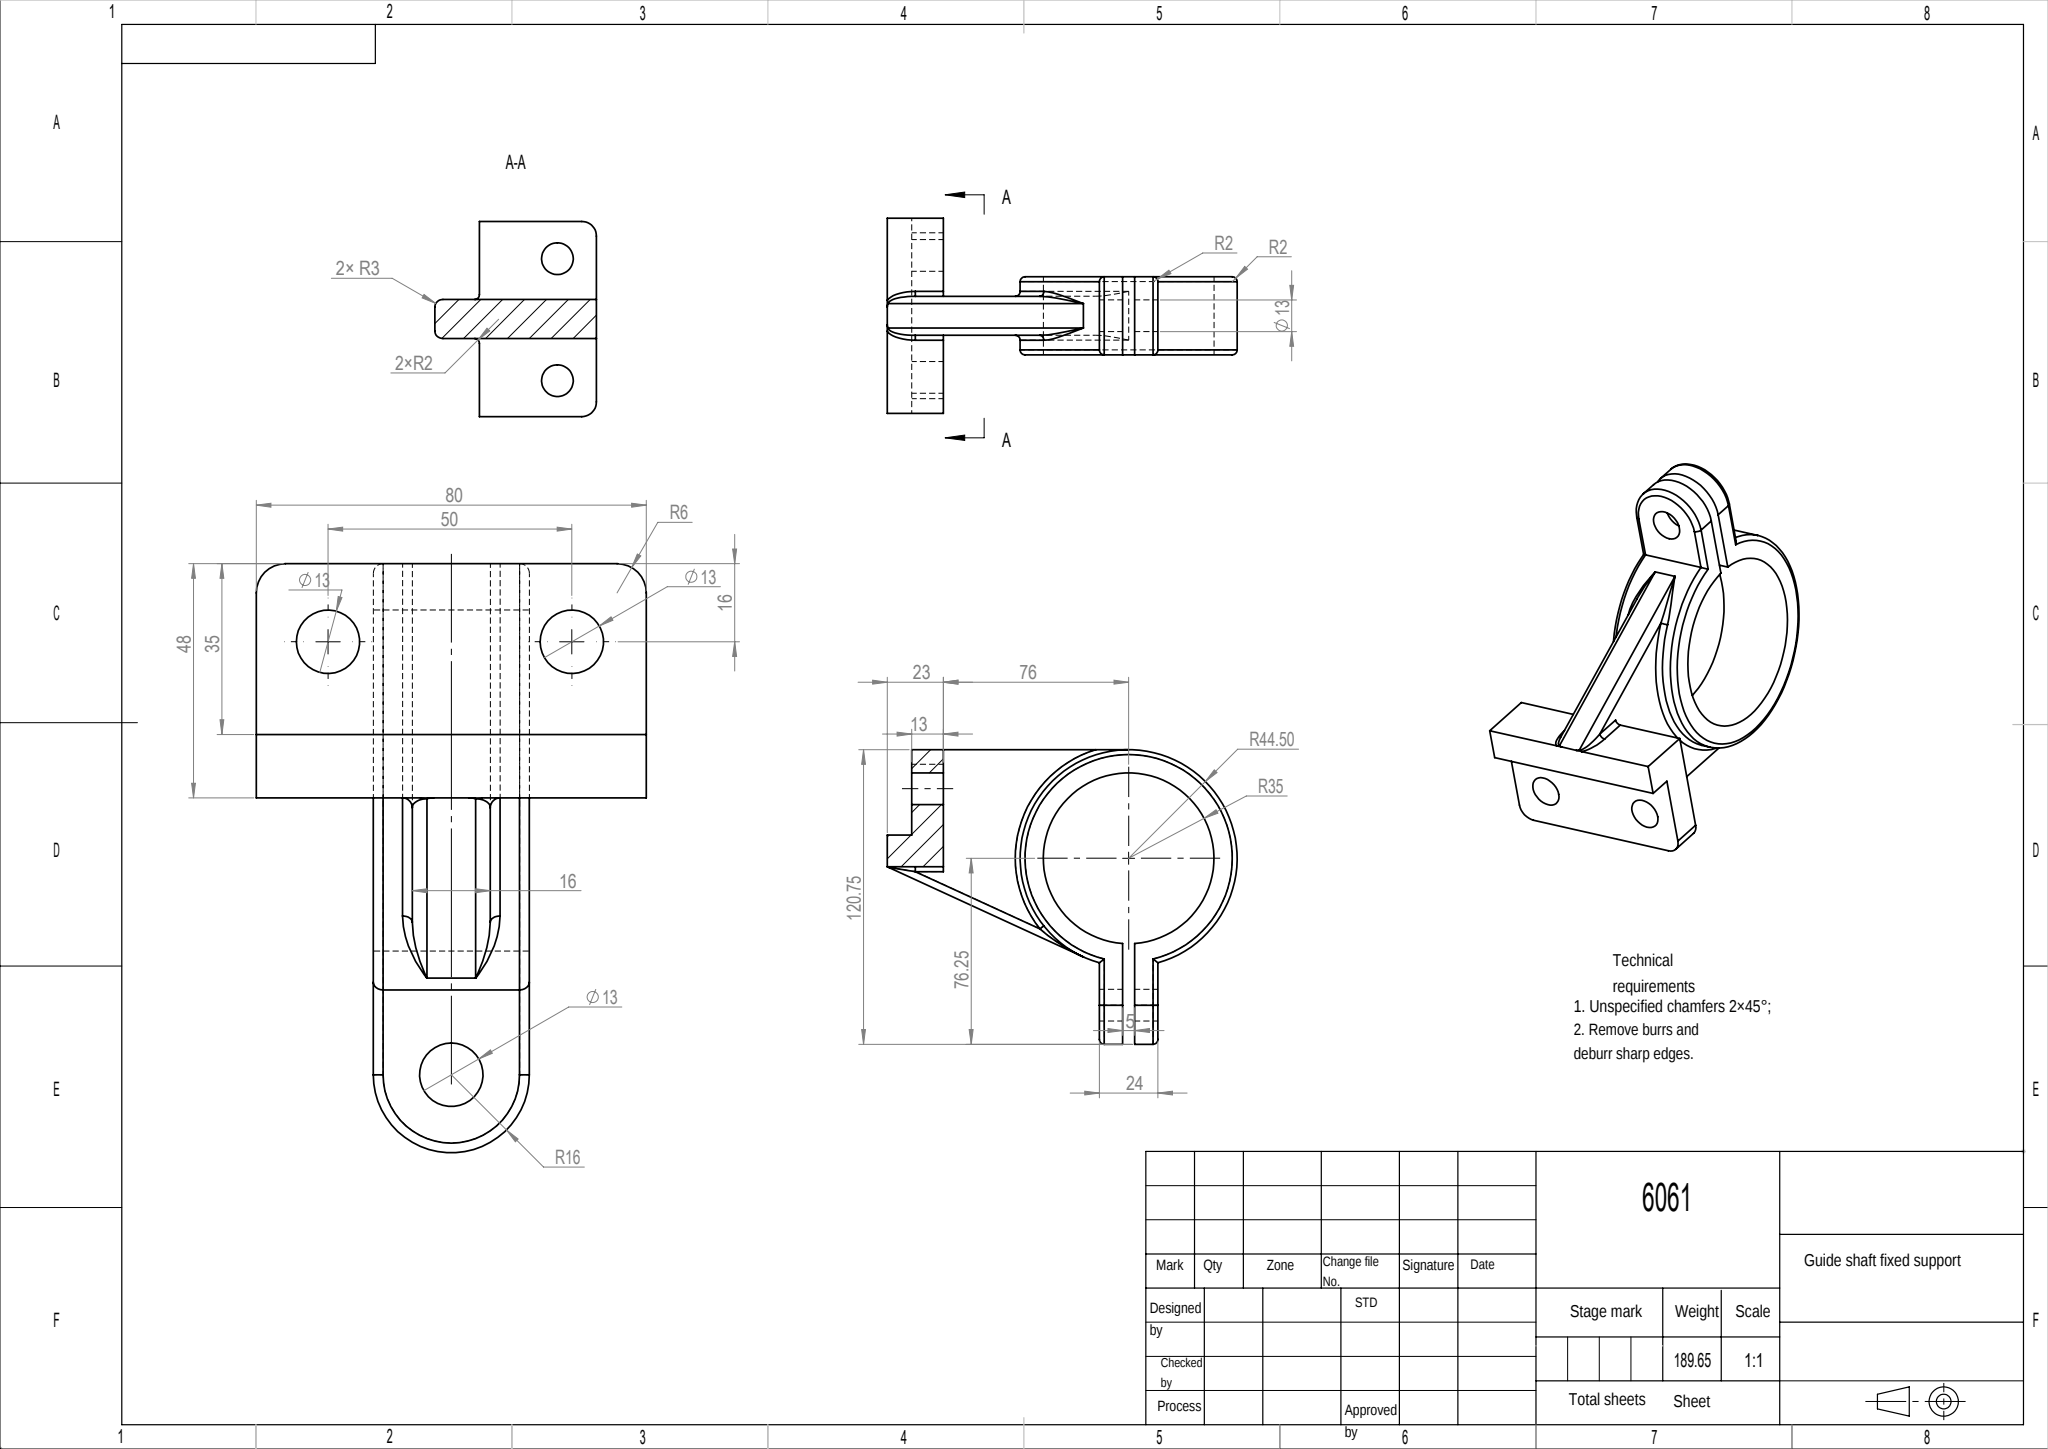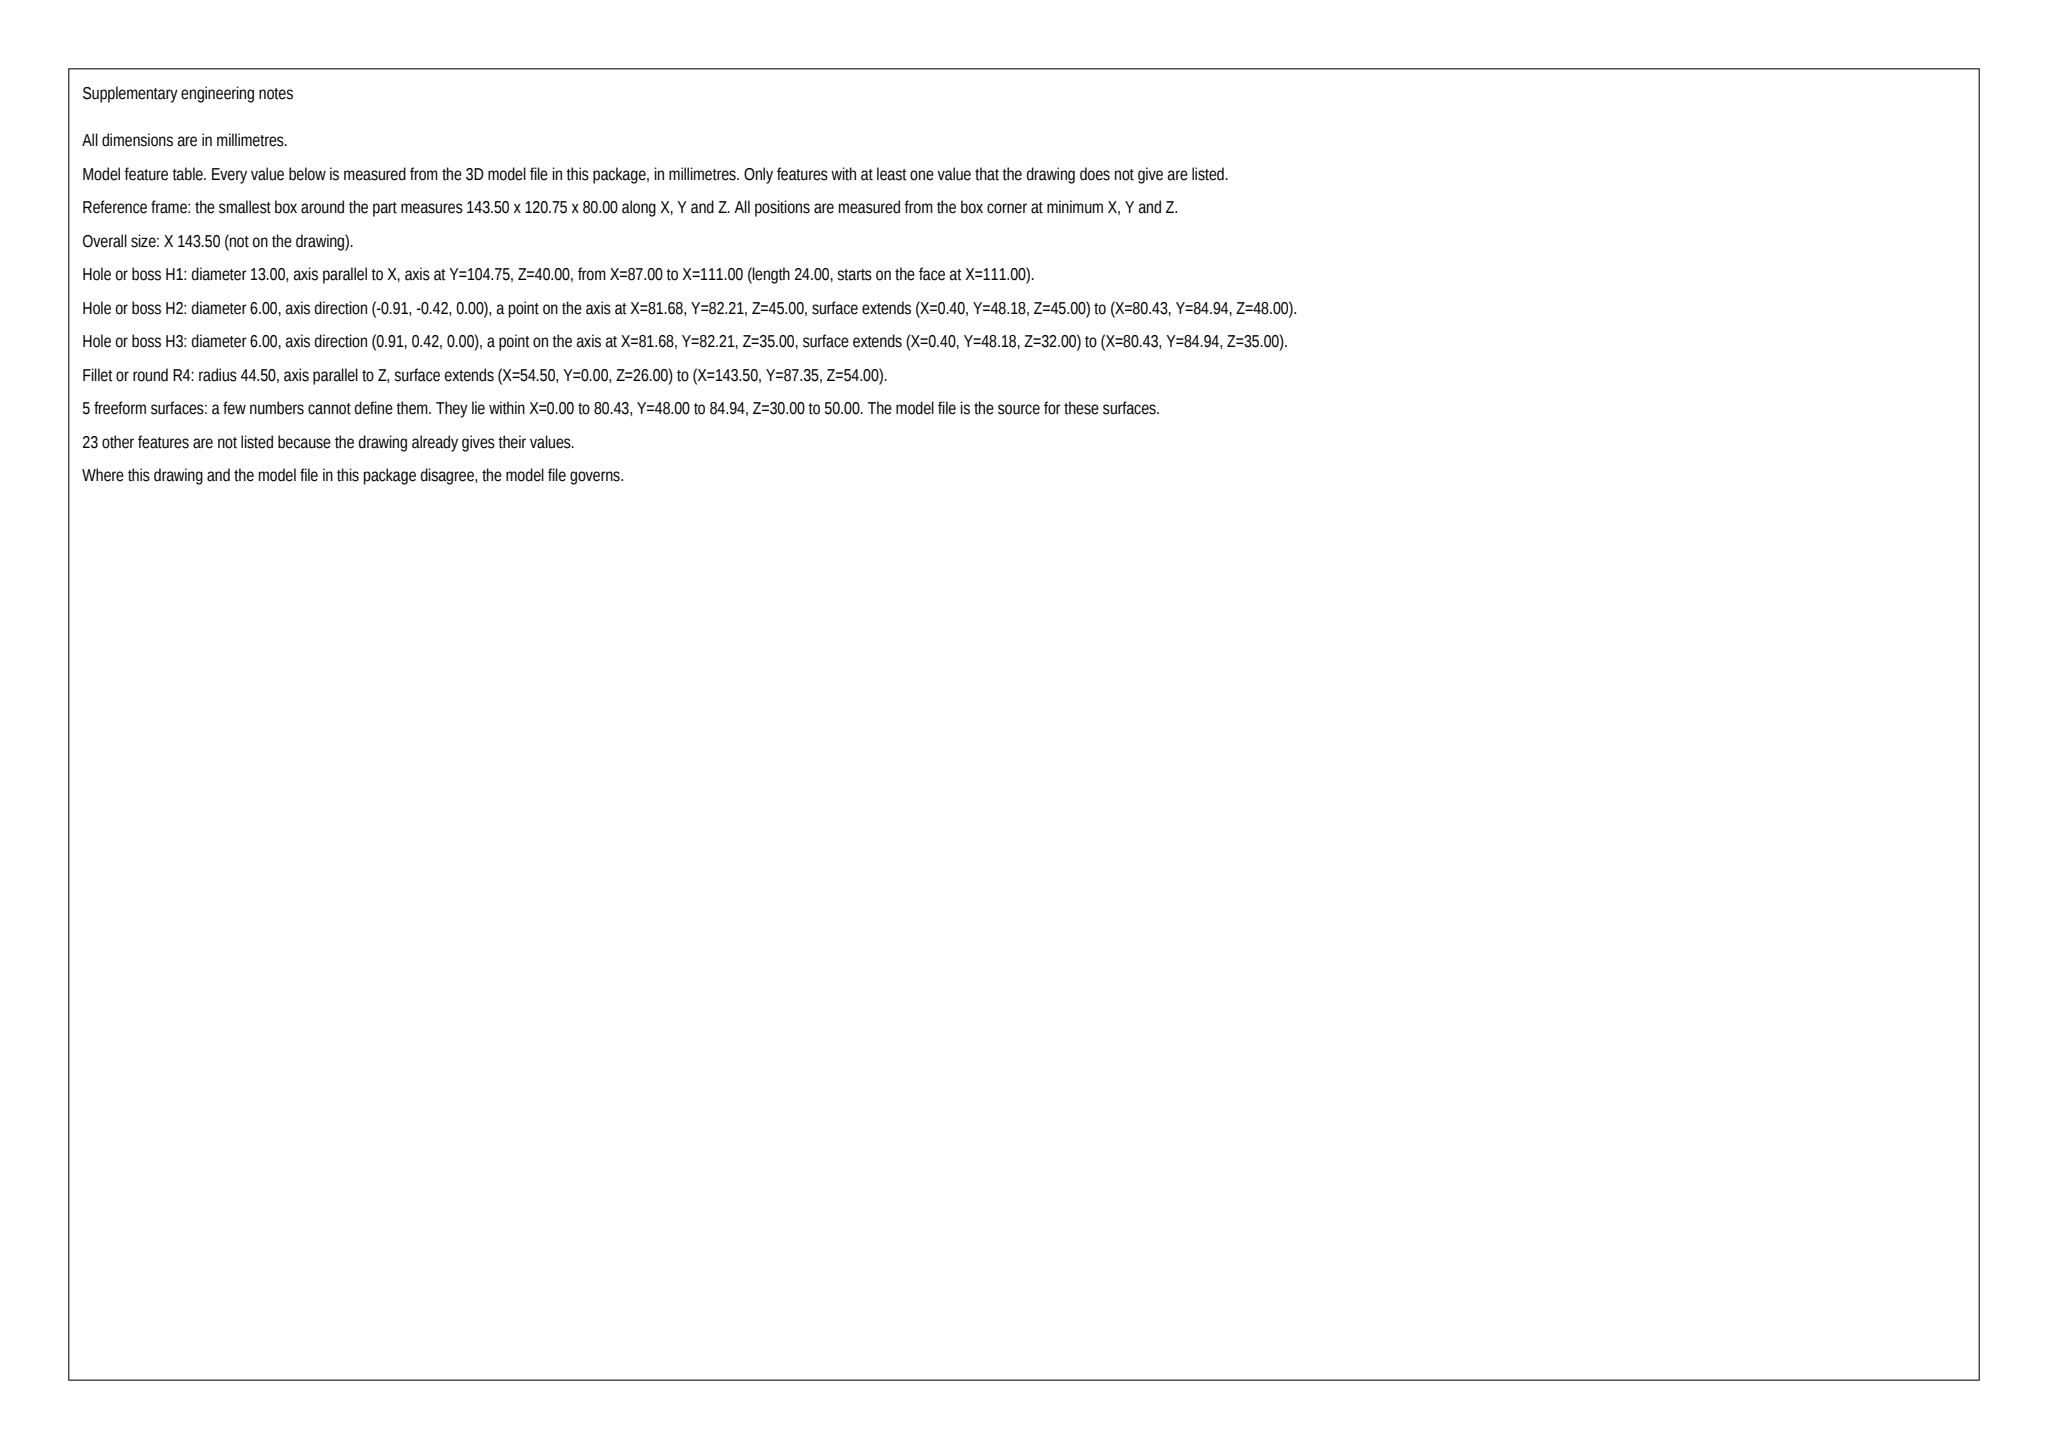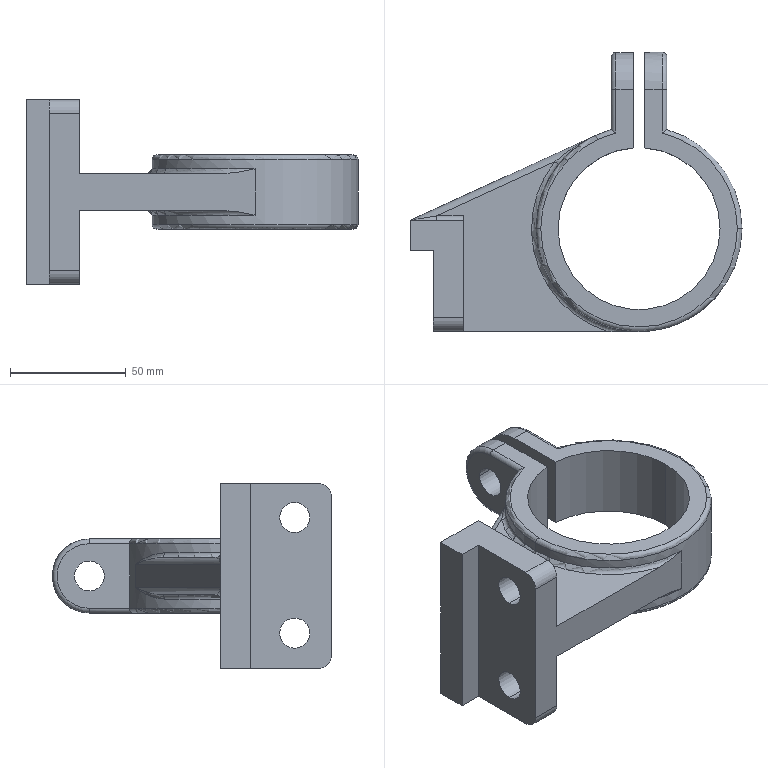Part | SolidWorks | mm | 1 solid | 61 faces | box 143.5 x 120.75 x 80 mm | volume 189650 mm3 | cylinder 26 | plane 19 | torus 11 | spline 5 | commonest cylinder face diameters 13 x8 4 x6 70 x3 89 x3 32 x2 12 x2 6 x2
Drawing notes:
OVERALL 147.64 x 129.44 x 80 | from the solid: bbox_xyz 147.636 x 129.438 x 80.001
BASE PLATE 13 THK; BTM STEP 23 THK x 13 HIGH, 10 PROUD OF PLATE FACE | from the solid: x-planes 0.47/10.47/23.47 (13 & 23 thk, 10 proud); y-planes 42.37/55.37 give 13 step
CLAMP RING 32 WIDE; Ø89 OD FACE 28 WIDE CTRD, R2 EA SIDE | from the solid: cyl Ø89 axis z len 28 at (99.47,51.87); ring Ø70 len 32; z-planes 24/32/48/56; fillet R2
Ø70 BORE (R35) THRU FULL 32 RING WIDTH | from the solid: cyl dia 70 axis z, pos (99.47,51.87), length 32
CLAMP SPLIT GAP 5; EARS 9.5 THK EA, 24 ACROSS, Ø13 THRU | from the solid: x-planes 87.47/96.97/101.97/111.47; Ø13 axis x len 9.5 x4 at y112.12 z40
RIB 16 THK CTRD ON RING AXIS PL; ROOT ON PLATE FACE, FLUSH W/ PLATE BTM EDGE | from the solid: z-planes 32 & 48 (16 ctrd on z=40 ring axis); rib root x=23.47 plate front face; plate y 7.37..55.37 = 48